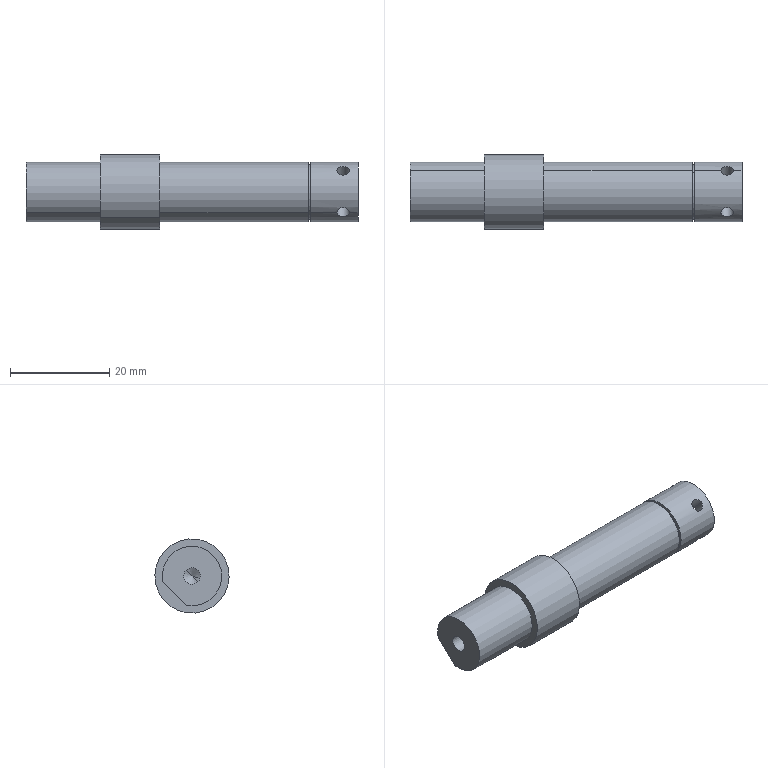Component | SolidWorks | ElectricalBoxAssembly2-1_AngleSensorComponentAssembly3-1_AngleSensorConnectionAxis-1 | 1 solid | 34 faces | box 67 x 15 x 15 mm | volume 7813 mm3 | cylinder 23 | plane 7 | cone 4 | commonest cylinder face diameters 2.5 x8 12 x7 6 x2 11 x2 3.3 x2 15 x2
build123d program:
from build123d import *

# Parameters (mm, degrees)
SKETCH1_R                     = 6
BOSS_EXTRUDE1_DEPTH           = 15
SKETCH2_R                     = 7.5
BOSS_EXTRUDE2_DEPTH           = 12
SKETCH3_R                     = 6
BOSS_EXTRUDE3_DEPTH           = 40
M4_TAPPED_HOLE1_D             = 3.3
M4_TAPPED_HOLE1_DEPTH         = 10.1
M4_TAPPED_HOLE1_TIP           = 0.9914
CUT_EXTRUDE1_DEPTH            = 15
SKETCH7_W                     = 0.5
SKETCH7_H                     = 0.5
SIZE_MM_DOWEL_PIN_HOLE1_D     = 6
SIZE_MM_DOWEL_PIN_HOLE1_DEPTH = 10.1
SIZE_MM_DOWEL_PIN_HOLE1_TIP   = 1.803
M3_TAPPED_HOLE1_D             = 2.5
CIRPATTERN1_COUNT             = 4


with BuildPart() as part:
    # Sketch1 → Boss-Extrude1 (new body)
    with BuildSketch(Plane.XY):
        Circle(SKETCH1_R)
    extrude(amount=BOSS_EXTRUDE1_DEPTH)

    # Sketch2 → Boss-Extrude2 (add)
    with BuildSketch(Plane.XY.offset(15)):
        Circle(SKETCH2_R)
    extrude(amount=BOSS_EXTRUDE2_DEPTH)

    # Sketch3 → Boss-Extrude3 (add)
    with BuildSketch(Plane.XY.offset(27)):
        Circle(SKETCH3_R)
    extrude(amount=BOSS_EXTRUDE3_DEPTH)

    # M4 Tapped Hole1
    with Locations(Plane(origin=(0, 0, 0), x_dir=(-1, 0, 0), z_dir=(0, 0, -1))):
        with Locations((0, 0)):
            Hole(M4_TAPPED_HOLE1_D / 2, depth=M4_TAPPED_HOLE1_DEPTH)
            with Locations((0, 0, -(M4_TAPPED_HOLE1_DEPTH + M4_TAPPED_HOLE1_TIP / 2))):  # 118° drill point
                Cone(0, M4_TAPPED_HOLE1_D / 2, M4_TAPPED_HOLE1_TIP, mode=Mode.SUBTRACT)

    # Sketch6 → Cut-Extrude1 (cut)
    with BuildSketch(Plane(origin=(0, 0, 0), x_dir=(-1, 0, 0), z_dir=(0, 0, -1))):
        with BuildLine():
            Line((-3.317, 5), (3.317, 5))
            ThreePointArc((3.317, 5), (0, 6), (-3.317, 5))
        make_face()
    extrude(amount=-CUT_EXTRUDE1_DEPTH, mode=Mode.SUBTRACT)

    # Sketch7 → Cut-Revolve1 (revolve, cut)
    with BuildSketch(Plane(origin=(0, 0, 0), x_dir=(0, 0, -1), z_dir=(1, 0, 0)), mode=Mode.PRIVATE) as cut_revolve1_sk:
        with Locations((-57.25, 5.75)):
            Rectangle(SKETCH7_W, SKETCH7_H)
    revolve(cut_revolve1_sk.sketch.rotate(Axis((0, 0, 67), (0, 0, -1)), 90), axis=Axis((0, 0, 67), (0, 0, -1)), mode=Mode.SUBTRACT)

    # Size mm Dowel Pin Hole1
    with Locations(Plane.XY.offset(67)):
        with Locations((0, 0)):
            Hole(SIZE_MM_DOWEL_PIN_HOLE1_D / 2, depth=SIZE_MM_DOWEL_PIN_HOLE1_DEPTH)
            with Locations((0, 0, -(SIZE_MM_DOWEL_PIN_HOLE1_DEPTH + SIZE_MM_DOWEL_PIN_HOLE1_TIP / 2))):  # 118° drill point
                Cone(0, SIZE_MM_DOWEL_PIN_HOLE1_D / 2, SIZE_MM_DOWEL_PIN_HOLE1_TIP, mode=Mode.SUBTRACT)

    # M3 Tapped Hole1 (through all)
    with Locations(Plane(origin=(0, 6, 0), x_dir=(1, 0, 0), z_dir=(0, 1, 0))):
        with Locations((0, -64)):
            m3_tapped_hole1 = Hole(M3_TAPPED_HOLE1_D / 2)

    # CirPattern1: M3 Tapped Hole1 ×4 about axis
    cirpattern1_axis = Axis((0, 0, 67), (0, 0, -1))
    for i in range(1, CIRPATTERN1_COUNT):
        add(m3_tapped_hole1.rotate(cirpattern1_axis, i * 360 / CIRPATTERN1_COUNT), mode=Mode.SUBTRACT)


solid = part.part

# Placed as in the assembly
solid = solid.moved(Location((782.115, 214.666, 1746.399), (-46.363, 90, 0)))